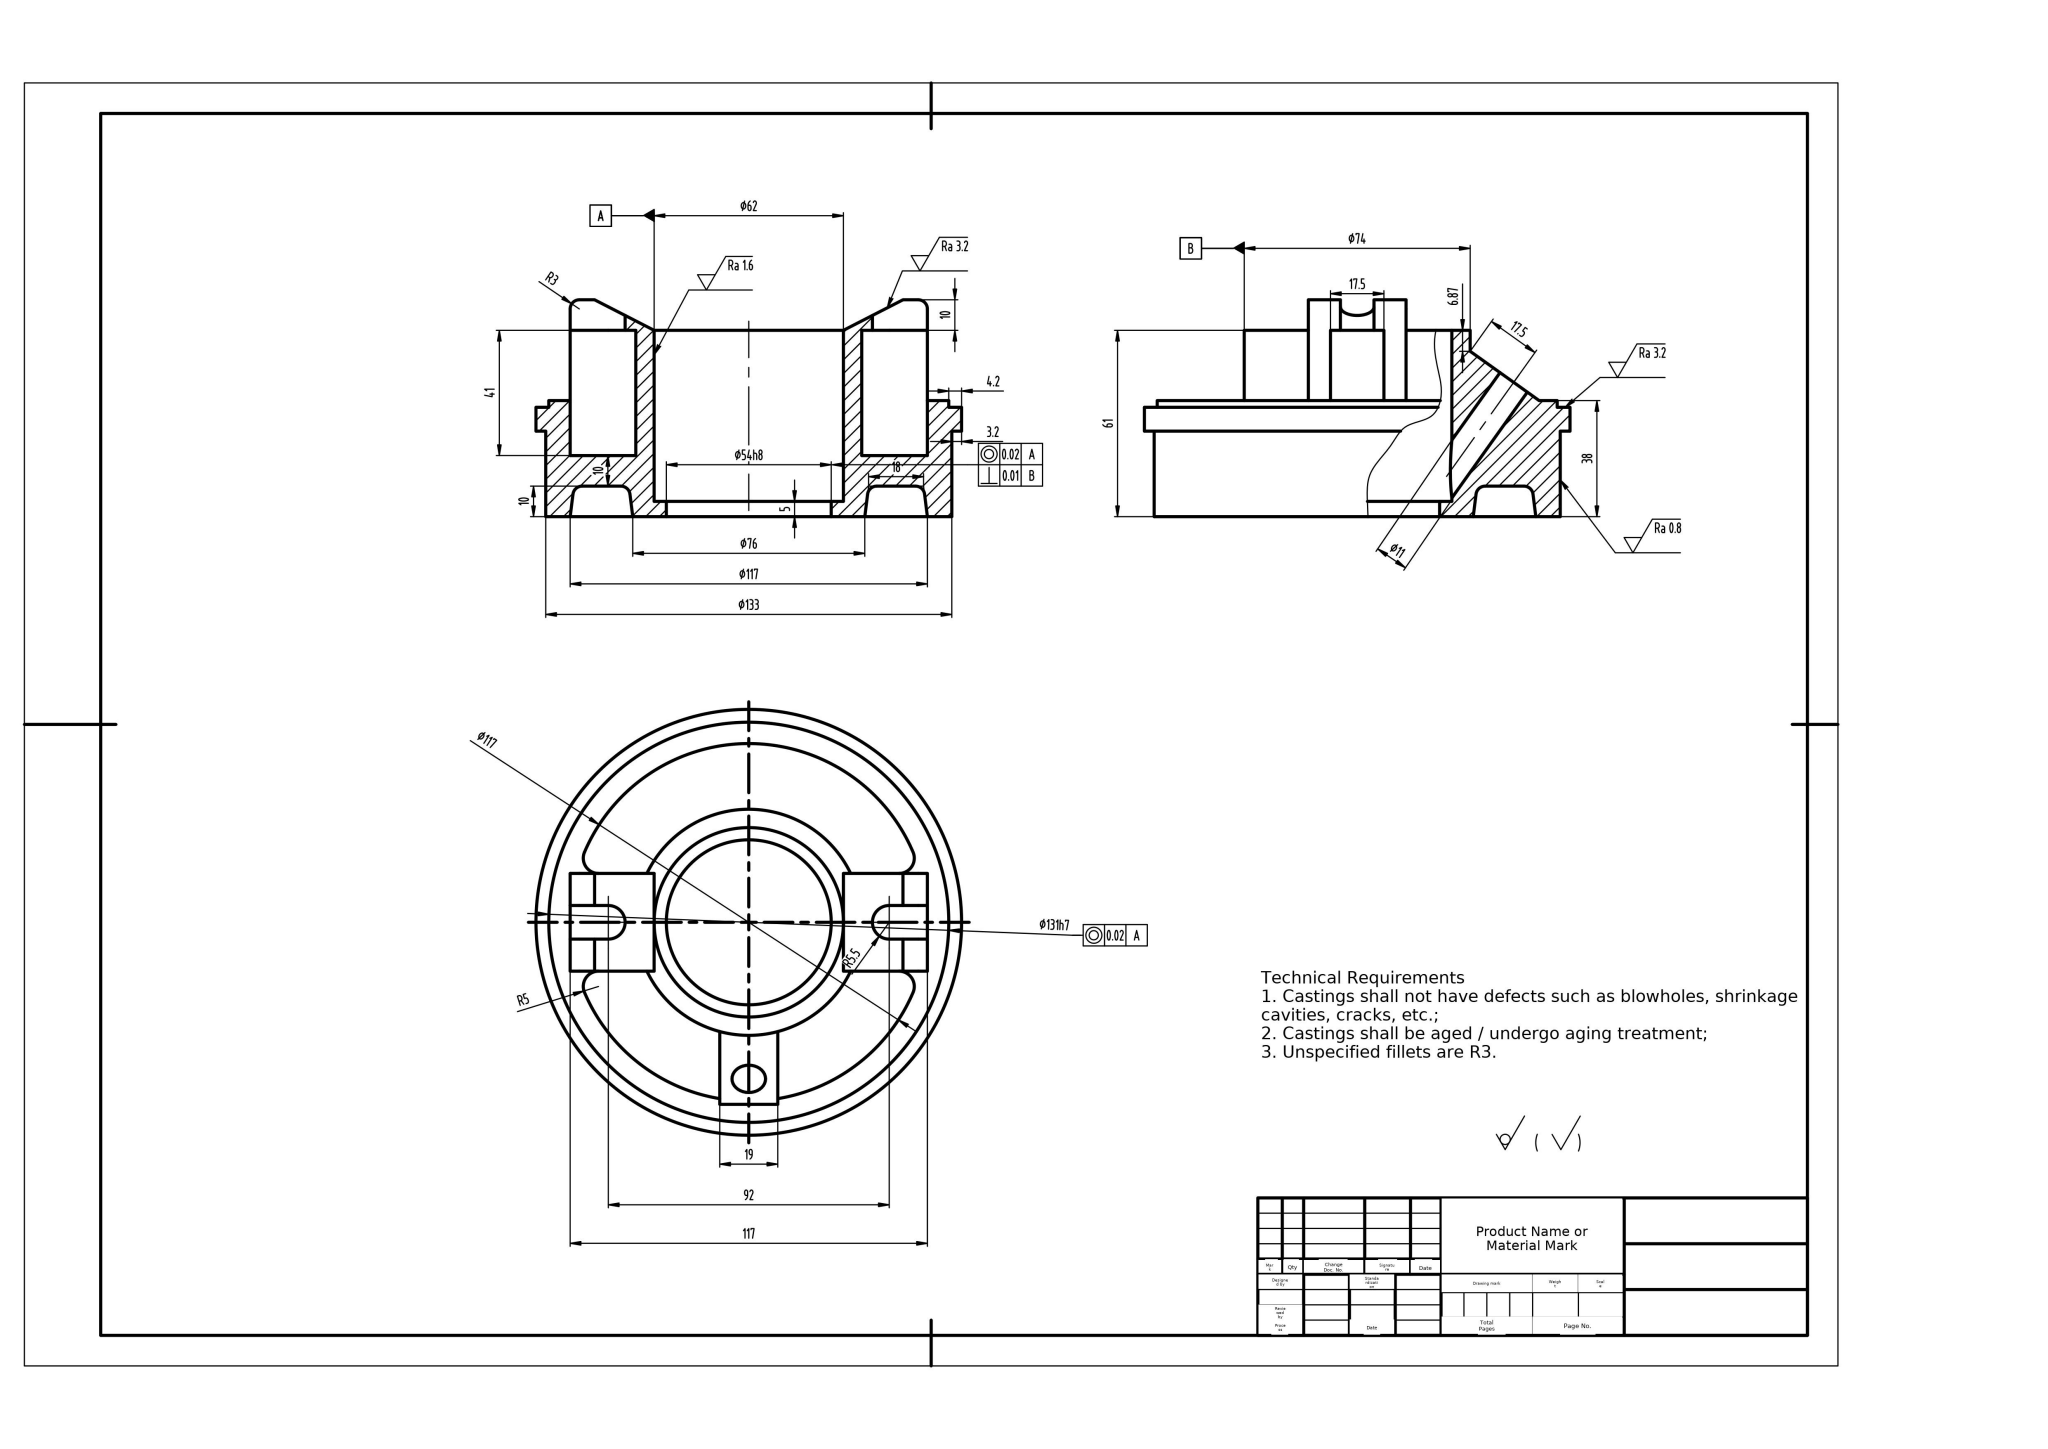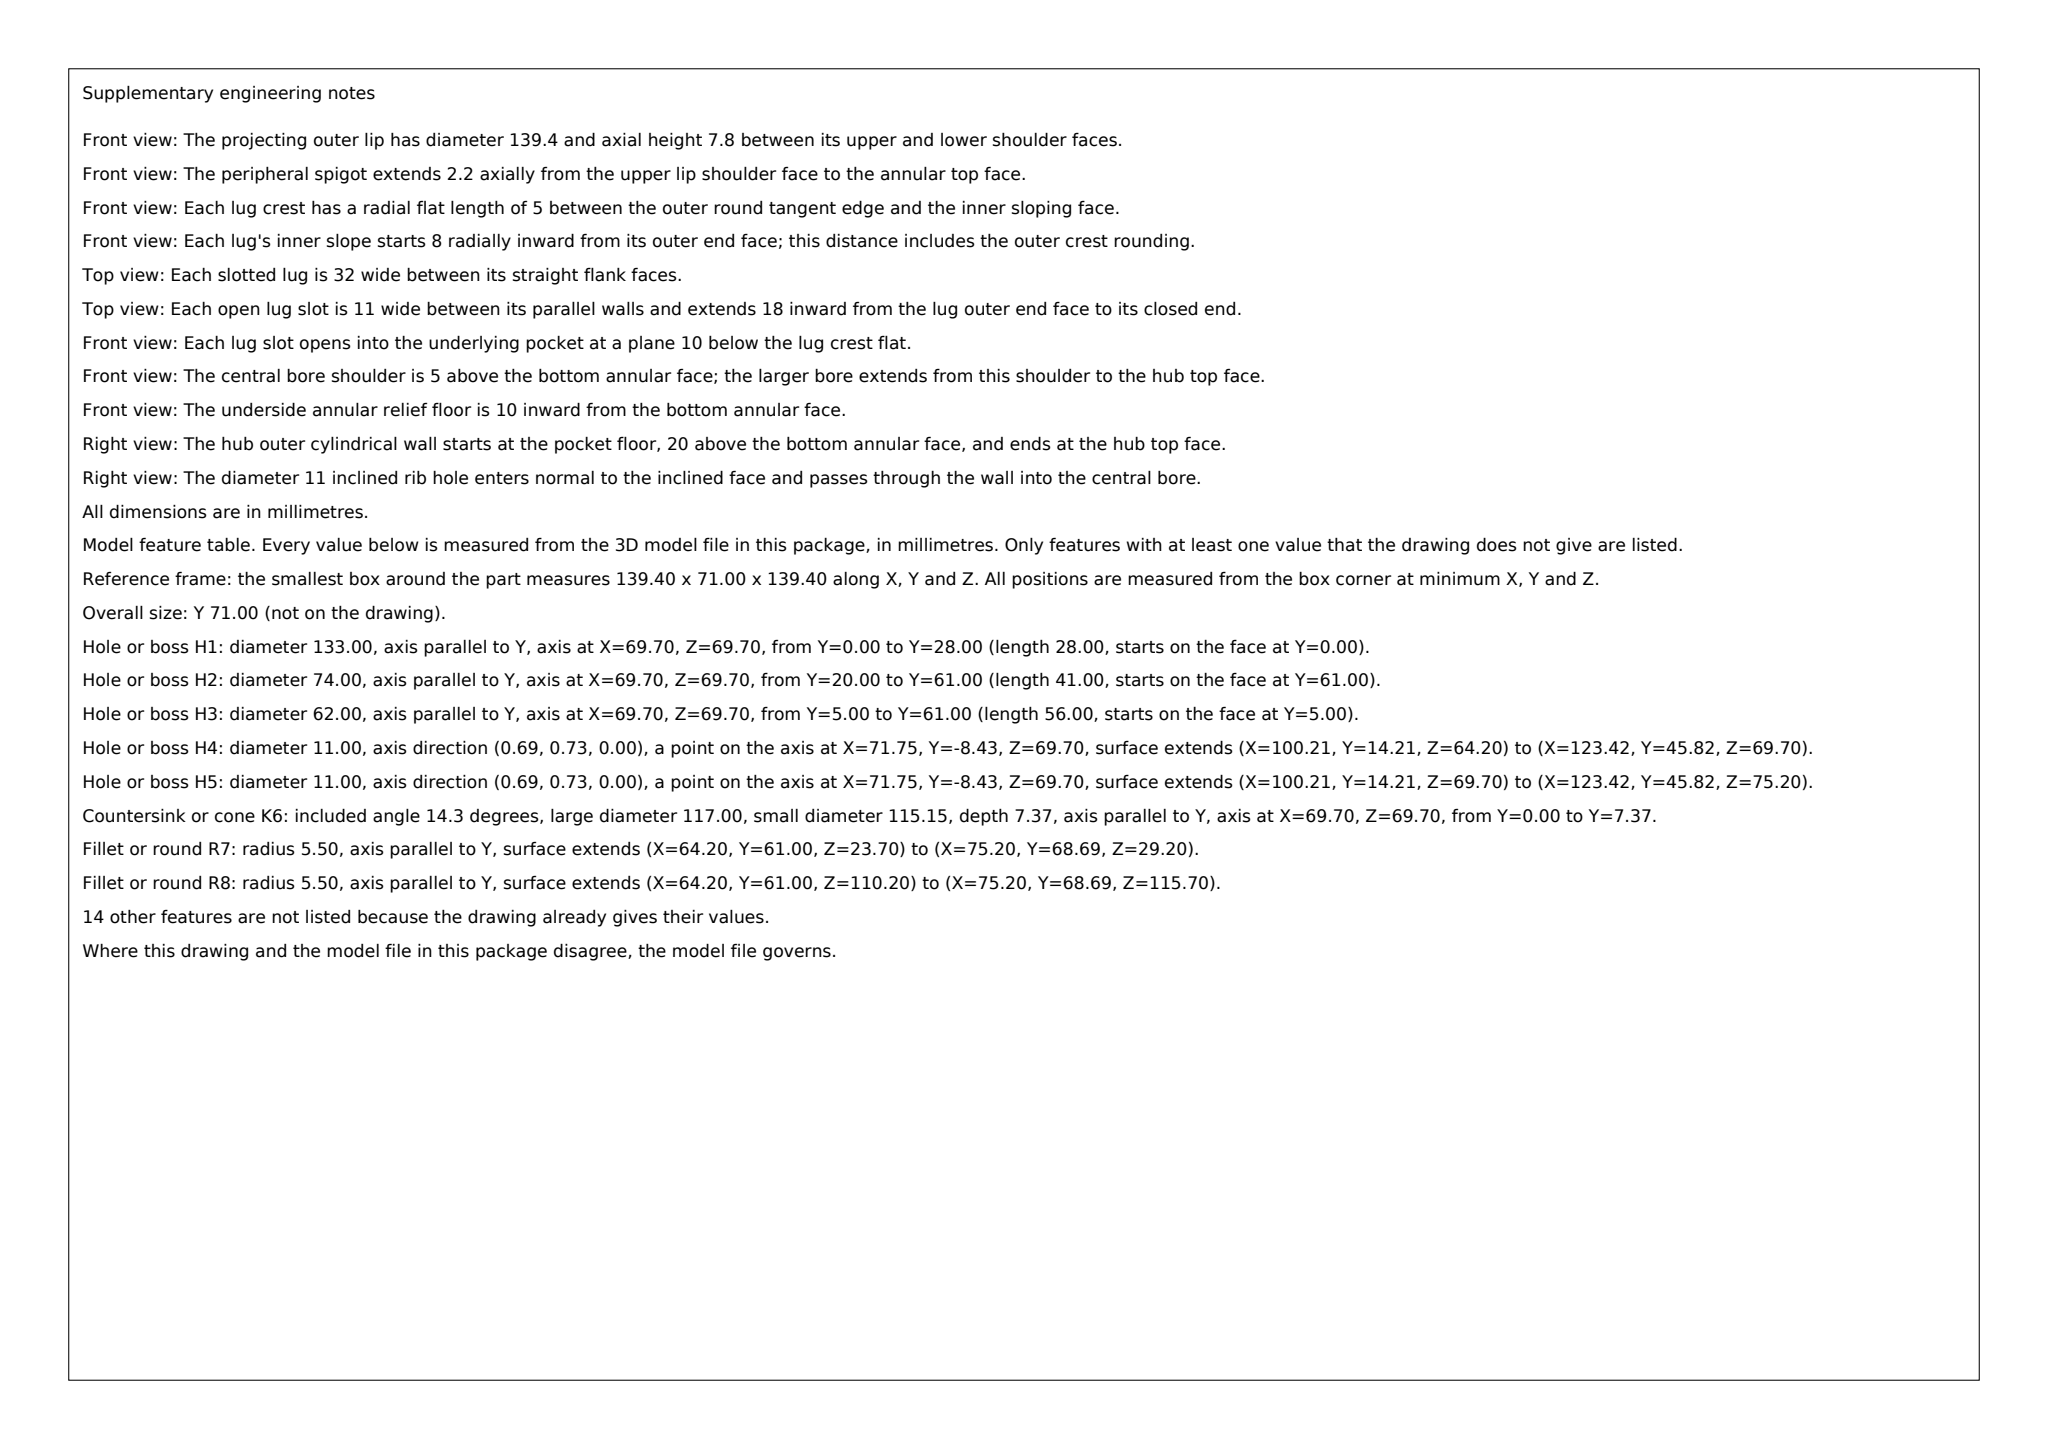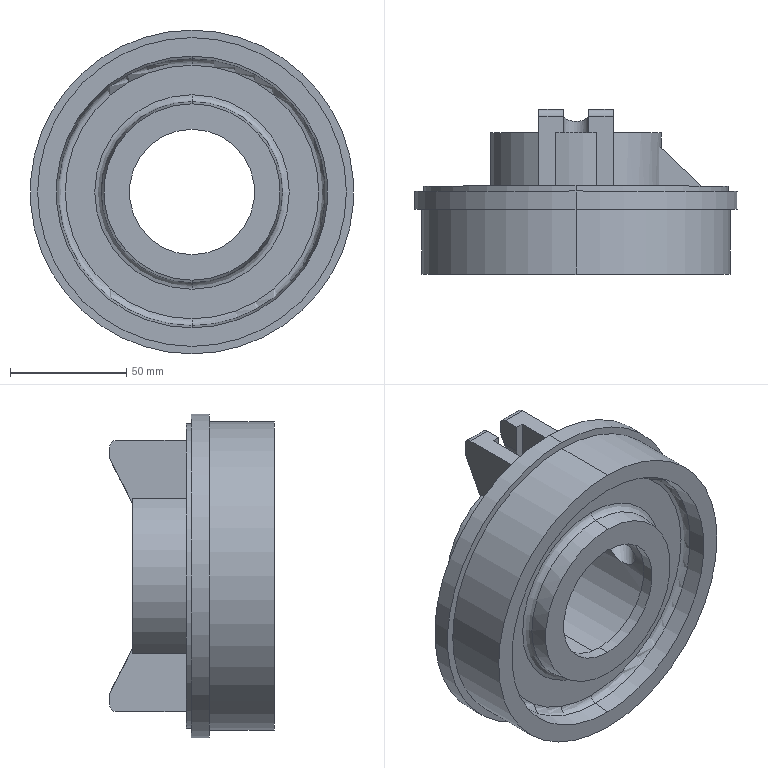Part | SolidWorks | mm | 1 solid | 84 faces | box 139.4 x 71 x 139.4 mm | volume 326240 mm3 | plane 43 | cylinder 33 | torus 4 | cone 4 | commonest cylinder face diameters 10 x6 11 x5 74 x5 6 x4 117 x3 131 x2 139.4 x2 133 x2
Drawing notes:
TOP LUG SLOT: 6 WIDE, R3 BOT, 6 DP FROM TOP FACE, 10.5 LG | from the solid: cyl Ø6 axis x at y=68, len 10.5 (x2); top face plane y=71 -> 71-(68-3)=6 deep
2 TOP LUGS: 55.5 EA SIDE OF AXIS C/L, 111 APART | from the solid: Ø6 slot cyls at z=14.2 & z=125.2; axis at z=69.7 -> 55.5 each side
FLANGE ARC SLOTS: Ø10 WIDE (R5) x 18 DP, R53.5, ENDS 21 FR C/L | from the solid: Ø10 axis-y cyls len 18 at (48.7,20.49)(48.7,118.91)(90.7,20.49)(90.7,118.91); axis 69.7,69.7 -> ±21, ±49.21, R=53.5
TAPERED (DRAFT) SURFS: 14.3° INCL ANGLE, REF Ø114.5 & Ø76 | from the solid: cones[14.3,114.5]x2 and cones[14.3,76]x2
Ø11 HOLE ON 43.4° BOSS: 31.6 DP ALONG HOLE AXIS | from the solid: cyl Ø11 at (x=71.75,z=69.7) length 31.61, only Ø11 on boss centreplane
2X Ø11 DP 7.7 THRU LUGS, 92 APART, SYM ABT DATUM A AXIS | from the solid: cyl dia 11, axis y, len 7.69 at (x=69.7, z=23.7) and (x=69.7, z=115.7); part axis at x=69.7, z=69.7 -> 46 each side = 92 apart